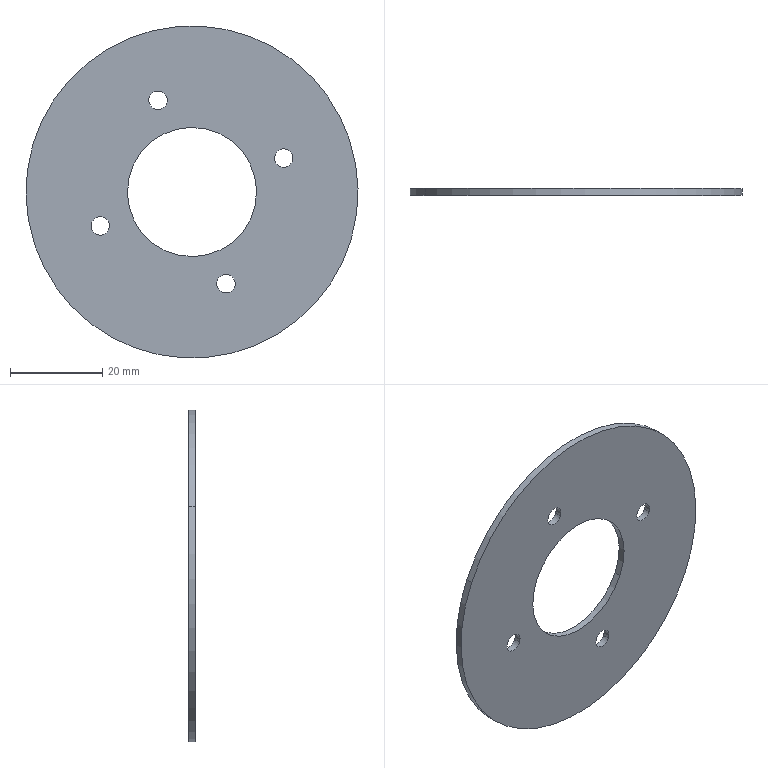Component | SolidWorks | Gear cover-1 | 1 solid | 14 faces | box 72 x 1.5 x 72 mm | volume 5108 mm3 | cylinder 12 | plane 2 | commonest cylinder face diameters 4 x8 28 x2 72 x2
STEP:
#1=COLOUR_RGB('',0.7922,0.8196,0.9333);
#2=FILL_AREA_STYLE_COLOUR('',#1);
#3=FILL_AREA_STYLE('',(#2));
#4=SURFACE_STYLE_FILL_AREA(#3);
#5=SURFACE_SIDE_STYLE('',(#4));
#6=SURFACE_STYLE_USAGE(.BOTH.,#5);
#7=PRESENTATION_STYLE_ASSIGNMENT((#6));
#8=CARTESIAN_POINT('',(-1.289,-1.213,-2.141));
#9=VERTEX_POINT('',#8);
#10=CARTESIAN_POINT('',(-1.146,-1.213,-2.207));
#11=VERTEX_POINT('',#10);
#12=CARTESIAN_POINT('',(-1.218,-1.213,-2.174));
#13=DIRECTION('',(-0.,-1.,0.));
#14=DIRECTION('',(0.9087,0.,-0.4174));
#15=AXIS2_PLACEMENT_3D('',#12,#13,#14);
#16=CIRCLE('',#15,0.07874);
#17=EDGE_CURVE('',#9,#11,#16,.T.);
#18=ORIENTED_EDGE('',*,*,#17,.T.);
#19=CARTESIAN_POINT('',(-1.146,-1.154,-2.207));
#20=VERTEX_POINT('',#19);
#21=CARTESIAN_POINT('',(-1.146,-1.213,-2.207));
#22=DIRECTION('',(0.,1.,-0.));
#23=VECTOR('',#22,39.37);
#24=LINE('',#21,#23);
#25=EDGE_CURVE('',#11,#20,#24,.T.);
#26=ORIENTED_EDGE('',*,*,#25,.T.);
#27=CARTESIAN_POINT('',(-1.289,-1.154,-2.141));
#28=VERTEX_POINT('',#27);
#29=CARTESIAN_POINT('',(-1.218,-1.154,-2.174));
#30=DIRECTION('',(-0.,-1.,0.));
#31=DIRECTION('',(0.9087,0.,-0.4174));
#32=AXIS2_PLACEMENT_3D('',#29,#30,#31);
#33=CIRCLE('',#32,0.07874);
#34=EDGE_CURVE('',#28,#20,#33,.T.);
#35=ORIENTED_EDGE('',*,*,#34,.F.);
#36=CARTESIAN_POINT('',(-1.289,-1.213,-2.141));
#37=DIRECTION('',(0.,1.,-0.));
#38=VECTOR('',#37,39.37);
#39=LINE('',#36,#38);
#40=EDGE_CURVE('',#9,#28,#39,.T.);
#41=ORIENTED_EDGE('',*,*,#40,.F.);
#42=EDGE_LOOP('',(#18,#26,#35,#41));
#43=FACE_OUTER_BOUND('',#42,.T.);
#44=CARTESIAN_POINT('',(-1.218,-1.213,-2.174));
#45=DIRECTION('',(0.,1.,-0.));
#46=DIRECTION('',(-0.9087,0.,0.4174));
#47=AXIS2_PLACEMENT_3D('',#44,#45,#46);
#48=CYLINDRICAL_SURFACE('',#47,0.07874);
#49=ADVANCED_FACE('',(#43),#48,.F.);
#50=CARTESIAN_POINT('',(-0.216,-1.213,-2.634));
#51=VERTEX_POINT('',#50);
#52=CARTESIAN_POINT('',(-0.0729,-1.213,-2.7));
#53=VERTEX_POINT('',#52);
#54=CARTESIAN_POINT('',(-0.1445,-1.213,-2.667));
#55=DIRECTION('',(-0.,-1.,0.));
#56=DIRECTION('',(0.9087,0.,-0.4174));
#57=AXIS2_PLACEMENT_3D('',#54,#55,#56);
#58=CIRCLE('',#57,0.07874);
#59=EDGE_CURVE('',#51,#53,#58,.T.);
#60=ORIENTED_EDGE('',*,*,#59,.T.);
#61=CARTESIAN_POINT('',(-0.0729,-1.154,-2.7));
#62=VERTEX_POINT('',#61);
#63=CARTESIAN_POINT('',(-0.0729,-1.213,-2.7));
#64=DIRECTION('',(0.,1.,-0.));
#65=VECTOR('',#64,39.37);
#66=LINE('',#63,#65);
#67=EDGE_CURVE('',#53,#62,#66,.T.);
#68=ORIENTED_EDGE('',*,*,#67,.T.);
#69=CARTESIAN_POINT('',(-0.216,-1.154,-2.634));
#70=VERTEX_POINT('',#69);
#71=CARTESIAN_POINT('',(-0.1445,-1.154,-2.667));
#72=DIRECTION('',(-0.,-1.,0.));
#73=DIRECTION('',(0.9087,0.,-0.4174));
#74=AXIS2_PLACEMENT_3D('',#71,#72,#73);
#75=CIRCLE('',#74,0.07874);
#76=EDGE_CURVE('',#70,#62,#75,.T.);
#77=ORIENTED_EDGE('',*,*,#76,.F.);
#78=CARTESIAN_POINT('',(-0.216,-1.213,-2.634));
#79=DIRECTION('',(0.,1.,-0.));
#80=VECTOR('',#79,39.37);
#81=LINE('',#78,#80);
#82=EDGE_CURVE('',#51,#70,#81,.T.);
#83=ORIENTED_EDGE('',*,*,#82,.F.);
#84=EDGE_LOOP('',(#60,#68,#77,#83));
#85=FACE_OUTER_BOUND('',#84,.T.);
#86=CARTESIAN_POINT('',(-0.1445,-1.213,-2.667));
#87=DIRECTION('',(0.,1.,-0.));
#88=DIRECTION('',(-0.9087,0.,0.4174));
#89=AXIS2_PLACEMENT_3D('',#86,#87,#88);
#90=CYLINDRICAL_SURFACE('',#89,0.07874);
#91=ADVANCED_FACE('',(#85),#90,.F.);
#92=CARTESIAN_POINT('',(0.277,-1.213,-1.561));
#93=VERTEX_POINT('',#92);
#94=CARTESIAN_POINT('',(0.4201,-1.213,-1.627));
#95=VERTEX_POINT('',#94);
#96=CARTESIAN_POINT('',(0.3486,-1.213,-1.594));
#97=DIRECTION('',(-0.,-1.,0.));
#98=DIRECTION('',(0.9087,0.,-0.4174));
#99=AXIS2_PLACEMENT_3D('',#96,#97,#98);
#100=CIRCLE('',#99,0.07874);
#101=EDGE_CURVE('',#93,#95,#100,.T.);
#102=ORIENTED_EDGE('',*,*,#101,.T.);
#103=CARTESIAN_POINT('',(0.4201,-1.154,-1.627));
#104=VERTEX_POINT('',#103);
#105=CARTESIAN_POINT('',(0.4201,-1.213,-1.627));
#106=DIRECTION('',(0.,1.,-0.));
#107=VECTOR('',#106,39.37);
#108=LINE('',#105,#107);
#109=EDGE_CURVE('',#95,#104,#108,.T.);
#110=ORIENTED_EDGE('',*,*,#109,.T.);
#111=CARTESIAN_POINT('',(0.277,-1.154,-1.561));
#112=VERTEX_POINT('',#111);
#113=CARTESIAN_POINT('',(0.3486,-1.154,-1.594));
#114=DIRECTION('',(-0.,-1.,0.));
#115=DIRECTION('',(0.9087,0.,-0.4174));
#116=AXIS2_PLACEMENT_3D('',#113,#114,#115);
#117=CIRCLE('',#116,0.07874);
#118=EDGE_CURVE('',#112,#104,#117,.T.);
#119=ORIENTED_EDGE('',*,*,#118,.F.);
#120=CARTESIAN_POINT('',(0.277,-1.213,-1.561));
#121=DIRECTION('',(0.,1.,-0.));
#122=VECTOR('',#121,39.37);
#123=LINE('',#120,#122);
#124=EDGE_CURVE('',#93,#112,#123,.T.);
#125=ORIENTED_EDGE('',*,*,#124,.F.);
#126=EDGE_LOOP('',(#102,#110,#119,#125));
#127=FACE_OUTER_BOUND('',#126,.T.);
#128=CARTESIAN_POINT('',(0.3486,-1.213,-1.594));
#129=DIRECTION('',(0.,1.,-0.));
#130=DIRECTION('',(-0.9087,0.,0.4174));
#131=AXIS2_PLACEMENT_3D('',#128,#129,#130);
#132=CYLINDRICAL_SURFACE('',#131,0.07874);
#133=ADVANCED_FACE('',(#127),#132,.F.);
#134=CARTESIAN_POINT('',(-0.7963,-1.213,-1.068));
#135=VERTEX_POINT('',#134);
#136=CARTESIAN_POINT('',(-0.6532,-1.213,-1.134));
#137=VERTEX_POINT('',#136);
#138=CARTESIAN_POINT('',(-0.7247,-1.213,-1.101));
#139=DIRECTION('',(-0.,-1.,0.));
#140=DIRECTION('',(0.9087,0.,-0.4174));
#141=AXIS2_PLACEMENT_3D('',#138,#139,#140);
#142=CIRCLE('',#141,0.07874);
#143=EDGE_CURVE('',#135,#137,#142,.T.);
#144=ORIENTED_EDGE('',*,*,#143,.T.);
#145=CARTESIAN_POINT('',(-0.6532,-1.154,-1.134));
#146=VERTEX_POINT('',#145);
#147=CARTESIAN_POINT('',(-0.6532,-1.213,-1.134));
#148=DIRECTION('',(0.,1.,-0.));
#149=VECTOR('',#148,39.37);
#150=LINE('',#147,#149);
#151=EDGE_CURVE('',#137,#146,#150,.T.);
#152=ORIENTED_EDGE('',*,*,#151,.T.);
#153=CARTESIAN_POINT('',(-0.7963,-1.154,-1.068));
#154=VERTEX_POINT('',#153);
#155=CARTESIAN_POINT('',(-0.7247,-1.154,-1.101));
#156=DIRECTION('',(-0.,-1.,0.));
#157=DIRECTION('',(0.9087,0.,-0.4174));
#158=AXIS2_PLACEMENT_3D('',#155,#156,#157);
#159=CIRCLE('',#158,0.07874);
#160=EDGE_CURVE('',#154,#146,#159,.T.);
#161=ORIENTED_EDGE('',*,*,#160,.F.);
#162=CARTESIAN_POINT('',(-0.7963,-1.213,-1.068));
#163=DIRECTION('',(0.,1.,-0.));
#164=VECTOR('',#163,39.37);
#165=LINE('',#162,#164);
#166=EDGE_CURVE('',#135,#154,#165,.T.);
#167=ORIENTED_EDGE('',*,*,#166,.F.);
#168=EDGE_LOOP('',(#144,#152,#161,#167));
#169=FACE_OUTER_BOUND('',#168,.T.);
#170=CARTESIAN_POINT('',(-0.7247,-1.213,-1.101));
#171=DIRECTION('',(0.,1.,-0.));
#172=DIRECTION('',(-0.9087,0.,0.4174));
#173=AXIS2_PLACEMENT_3D('',#170,#171,#172);
#174=CYLINDRICAL_SURFACE('',#173,0.07874);
#175=ADVANCED_FACE('',(#169),#174,.F.);
#176=CARTESIAN_POINT('',(-0.9354,-1.213,-1.654));
#177=VERTEX_POINT('',#176);
#178=CARTESIAN_POINT('',(0.06628,-1.213,-2.114));
#179=VERTEX_POINT('',#178);
#180=CARTESIAN_POINT('',(-0.4346,-1.213,-1.884));
#181=DIRECTION('',(-0.,-1.,0.));
#182=DIRECTION('',(0.9087,-0.,-0.4174));
#183=AXIS2_PLACEMENT_3D('',#180,#181,#182);
#184=CIRCLE('',#183,0.5512);
#185=EDGE_CURVE('',#177,#179,#184,.T.);
#186=ORIENTED_EDGE('',*,*,#185,.T.);
#187=CARTESIAN_POINT('',(0.06628,-1.154,-2.114));
#188=VERTEX_POINT('',#187);
#189=CARTESIAN_POINT('',(0.06628,-1.213,-2.114));
#190=DIRECTION('',(0.,1.,-0.));
#191=VECTOR('',#190,39.37);
#192=LINE('',#189,#191);
#193=EDGE_CURVE('',#179,#188,#192,.T.);
#194=ORIENTED_EDGE('',*,*,#193,.T.);
#195=CARTESIAN_POINT('',(-0.9354,-1.154,-1.654));
#196=VERTEX_POINT('',#195);
#197=CARTESIAN_POINT('',(-0.4346,-1.154,-1.884));
#198=DIRECTION('',(-0.,-1.,0.));
#199=DIRECTION('',(0.9087,-0.,-0.4174));
#200=AXIS2_PLACEMENT_3D('',#197,#198,#199);
#201=CIRCLE('',#200,0.5512);
#202=EDGE_CURVE('',#196,#188,#201,.T.);
#203=ORIENTED_EDGE('',*,*,#202,.F.);
#204=CARTESIAN_POINT('',(-0.9354,-1.213,-1.654));
#205=DIRECTION('',(0.,1.,-0.));
#206=VECTOR('',#205,39.37);
#207=LINE('',#204,#206);
#208=EDGE_CURVE('',#177,#196,#207,.T.);
#209=ORIENTED_EDGE('',*,*,#208,.F.);
#210=EDGE_LOOP('',(#186,#194,#203,#209));
#211=FACE_OUTER_BOUND('',#210,.T.);
#212=CARTESIAN_POINT('',(-0.4346,-1.213,-1.884));
#213=DIRECTION('',(0.,1.,-0.));
#214=DIRECTION('',(-0.9087,0.,0.4174));
#215=AXIS2_PLACEMENT_3D('',#212,#213,#214);
#216=CYLINDRICAL_SURFACE('',#215,0.5512);
#217=ADVANCED_FACE('',(#211),#216,.F.);
#218=CARTESIAN_POINT('',(0.8534,-1.213,-2.476));
#219=VERTEX_POINT('',#218);
#220=CARTESIAN_POINT('',(-1.723,-1.213,-1.292));
#221=VERTEX_POINT('',#220);
#222=CARTESIAN_POINT('',(-0.4346,-1.213,-1.884));
#223=DIRECTION('',(-0.,-1.,0.));
#224=DIRECTION('',(0.9087,-0.,-0.4174));
#225=AXIS2_PLACEMENT_3D('',#222,#223,#224);
#226=CIRCLE('',#225,1.417);
#227=EDGE_CURVE('',#219,#221,#226,.T.);
#228=ORIENTED_EDGE('',*,*,#227,.F.);
#229=CARTESIAN_POINT('',(0.8534,-1.154,-2.476));
#230=VERTEX_POINT('',#229);
#231=CARTESIAN_POINT('',(0.8534,-1.213,-2.476));
#232=DIRECTION('',(0.,1.,-0.));
#233=VECTOR('',#232,39.37);
#234=LINE('',#231,#233);
#235=EDGE_CURVE('',#219,#230,#234,.T.);
#236=ORIENTED_EDGE('',*,*,#235,.T.);
#237=CARTESIAN_POINT('',(-1.723,-1.154,-1.292));
#238=VERTEX_POINT('',#237);
#239=CARTESIAN_POINT('',(-0.4346,-1.154,-1.884));
#240=DIRECTION('',(-0.,-1.,0.));
#241=DIRECTION('',(0.9087,-0.,-0.4174));
#242=AXIS2_PLACEMENT_3D('',#239,#240,#241);
#243=CIRCLE('',#242,1.417);
#244=EDGE_CURVE('',#230,#238,#243,.T.);
#245=ORIENTED_EDGE('',*,*,#244,.T.);
#246=CARTESIAN_POINT('',(-1.723,-1.213,-1.292));
#247=DIRECTION('',(0.,1.,-0.));
#248=VECTOR('',#247,39.37);
#249=LINE('',#246,#248);
#250=EDGE_CURVE('',#221,#238,#249,.T.);
#251=ORIENTED_EDGE('',*,*,#250,.F.);
#252=EDGE_LOOP('',(#228,#236,#245,#251));
#253=FACE_OUTER_BOUND('',#252,.T.);
#254=CARTESIAN_POINT('',(-0.4346,-1.213,-1.884));
#255=DIRECTION('',(0.,1.,-0.));
#256=DIRECTION('',(-0.9087,0.,0.4174));
#257=AXIS2_PLACEMENT_3D('',#254,#255,#256);
#258=CYLINDRICAL_SURFACE('',#257,1.417);
#259=ADVANCED_FACE('',(#253),#258,.T.);
#260=ORIENTED_EDGE('',*,*,#59,.F.);
#261=CARTESIAN_POINT('',(-0.1445,-1.213,-2.667));
#262=DIRECTION('',(-0.,-1.,0.));
#263=DIRECTION('',(0.9087,0.,-0.4174));
#264=AXIS2_PLACEMENT_3D('',#261,#262,#263);
#265=CIRCLE('',#264,0.07874);
#266=EDGE_CURVE('',#53,#51,#265,.T.);
#267=ORIENTED_EDGE('',*,*,#266,.F.);
#268=EDGE_LOOP('',(#260,#267));
#269=FACE_BOUND('',#268,.T.);
#270=ORIENTED_EDGE('',*,*,#143,.F.);
#271=CARTESIAN_POINT('',(-0.7247,-1.213,-1.101));
#272=DIRECTION('',(-0.,-1.,0.));
#273=DIRECTION('',(0.9087,0.,-0.4174));
#274=AXIS2_PLACEMENT_3D('',#271,#272,#273);
#275=CIRCLE('',#274,0.07874);
#276=EDGE_CURVE('',#137,#135,#275,.T.);
#277=ORIENTED_EDGE('',*,*,#276,.F.);
#278=EDGE_LOOP('',(#270,#277));
#279=FACE_BOUND('',#278,.T.);
#280=CARTESIAN_POINT('',(-0.4346,-1.213,-1.884));
#281=DIRECTION('',(-0.,-1.,0.));
#282=DIRECTION('',(0.9087,-0.,-0.4174));
#283=AXIS2_PLACEMENT_3D('',#280,#281,#282);
#284=CIRCLE('',#283,1.417);
#285=EDGE_CURVE('',#221,#219,#284,.T.);
#286=ORIENTED_EDGE('',*,*,#285,.T.);
#287=ORIENTED_EDGE('',*,*,#227,.T.);
#288=EDGE_LOOP('',(#286,#287));
#289=FACE_OUTER_BOUND('',#288,.T.);
#290=ORIENTED_EDGE('',*,*,#185,.F.);
#291=CARTESIAN_POINT('',(-0.4346,-1.213,-1.884));
#292=DIRECTION('',(-0.,-1.,0.));
#293=DIRECTION('',(0.9087,-0.,-0.4174));
#294=AXIS2_PLACEMENT_3D('',#291,#292,#293);
#295=CIRCLE('',#294,0.5512);
#296=EDGE_CURVE('',#179,#177,#295,.T.);
#297=ORIENTED_EDGE('',*,*,#296,.F.);
#298=EDGE_LOOP('',(#290,#297));
#299=FACE_BOUND('',#298,.T.);
#300=ORIENTED_EDGE('',*,*,#101,.F.);
#301=CARTESIAN_POINT('',(0.3486,-1.213,-1.594));
#302=DIRECTION('',(-0.,-1.,0.));
#303=DIRECTION('',(0.9087,0.,-0.4174));
#304=AXIS2_PLACEMENT_3D('',#301,#302,#303);
#305=CIRCLE('',#304,0.07874);
#306=EDGE_CURVE('',#95,#93,#305,.T.);
#307=ORIENTED_EDGE('',*,*,#306,.F.);
#308=EDGE_LOOP('',(#300,#307));
#309=FACE_BOUND('',#308,.T.);
#310=ORIENTED_EDGE('',*,*,#17,.F.);
#311=CARTESIAN_POINT('',(-1.218,-1.213,-2.174));
#312=DIRECTION('',(-0.,-1.,0.));
#313=DIRECTION('',(0.9087,0.,-0.4174));
#314=AXIS2_PLACEMENT_3D('',#311,#312,#313);
#315=CIRCLE('',#314,0.07874);
#316=EDGE_CURVE('',#11,#9,#315,.T.);
#317=ORIENTED_EDGE('',*,*,#316,.F.);
#318=EDGE_LOOP('',(#310,#317));
#319=FACE_BOUND('',#318,.T.);
#320=CARTESIAN_POINT('',(-0.4346,-1.213,-1.884));
#321=DIRECTION('',(-0.,-1.,0.));
#322=DIRECTION('',(0.9087,-0.,-0.4174));
#323=AXIS2_PLACEMENT_3D('',#320,#321,#322);
#324=PLANE('',#323);
#325=ADVANCED_FACE('',(#269,#279,#289,#299,#309,#319),#324,.T.);
#326=ORIENTED_EDGE('',*,*,#76,.T.);
#327=CARTESIAN_POINT('',(-0.1445,-1.154,-2.667));
#328=DIRECTION('',(-0.,-1.,0.));
#329=DIRECTION('',(0.9087,0.,-0.4174));
#330=AXIS2_PLACEMENT_3D('',#327,#328,#329);
#331=CIRCLE('',#330,0.07874);
#332=EDGE_CURVE('',#62,#70,#331,.T.);
#333=ORIENTED_EDGE('',*,*,#332,.T.);
#334=EDGE_LOOP('',(#326,#333));
#335=FACE_BOUND('',#334,.T.);
#336=ORIENTED_EDGE('',*,*,#160,.T.);
#337=CARTESIAN_POINT('',(-0.7247,-1.154,-1.101));
#338=DIRECTION('',(-0.,-1.,0.));
#339=DIRECTION('',(0.9087,0.,-0.4174));
#340=AXIS2_PLACEMENT_3D('',#337,#338,#339);
#341=CIRCLE('',#340,0.07874);
#342=EDGE_CURVE('',#146,#154,#341,.T.);
#343=ORIENTED_EDGE('',*,*,#342,.T.);
#344=EDGE_LOOP('',(#336,#343));
#345=FACE_BOUND('',#344,.T.);
#346=CARTESIAN_POINT('',(-0.4346,-1.154,-1.884));
#347=DIRECTION('',(-0.,-1.,0.));
#348=DIRECTION('',(0.9087,-0.,-0.4174));
#349=AXIS2_PLACEMENT_3D('',#346,#347,#348);
#350=CIRCLE('',#349,1.417);
#351=EDGE_CURVE('',#238,#230,#350,.T.);
#352=ORIENTED_EDGE('',*,*,#351,.F.);
#353=ORIENTED_EDGE('',*,*,#244,.F.);
#354=EDGE_LOOP('',(#352,#353));
#355=FACE_OUTER_BOUND('',#354,.T.);
#356=ORIENTED_EDGE('',*,*,#202,.T.);
#357=CARTESIAN_POINT('',(-0.4346,-1.154,-1.884));
#358=DIRECTION('',(-0.,-1.,0.));
#359=DIRECTION('',(0.9087,-0.,-0.4174));
#360=AXIS2_PLACEMENT_3D('',#357,#358,#359);
#361=CIRCLE('',#360,0.5512);
#362=EDGE_CURVE('',#188,#196,#361,.T.);
#363=ORIENTED_EDGE('',*,*,#362,.T.);
#364=EDGE_LOOP('',(#356,#363));
#365=FACE_BOUND('',#364,.T.);
#366=ORIENTED_EDGE('',*,*,#118,.T.);
#367=CARTESIAN_POINT('',(0.3486,-1.154,-1.594));
#368=DIRECTION('',(-0.,-1.,0.));
#369=DIRECTION('',(0.9087,0.,-0.4174));
#370=AXIS2_PLACEMENT_3D('',#367,#368,#369);
#371=CIRCLE('',#370,0.07874);
#372=EDGE_CURVE('',#104,#112,#371,.T.);
#373=ORIENTED_EDGE('',*,*,#372,.T.);
#374=EDGE_LOOP('',(#366,#373));
#375=FACE_BOUND('',#374,.T.);
#376=ORIENTED_EDGE('',*,*,#34,.T.);
#377=CARTESIAN_POINT('',(-1.218,-1.154,-2.174));
#378=DIRECTION('',(-0.,-1.,0.));
#379=DIRECTION('',(0.9087,0.,-0.4174));
#380=AXIS2_PLACEMENT_3D('',#377,#378,#379);
#381=CIRCLE('',#380,0.07874);
#382=EDGE_CURVE('',#20,#28,#381,.T.);
#383=ORIENTED_EDGE('',*,*,#382,.T.);
#384=EDGE_LOOP('',(#376,#383));
#385=FACE_BOUND('',#384,.T.);
#386=CARTESIAN_POINT('',(-0.4346,-1.154,-1.884));
#387=DIRECTION('',(-0.,-1.,0.));
#388=DIRECTION('',(0.9087,-0.,-0.4174));
#389=AXIS2_PLACEMENT_3D('',#386,#387,#388);
#390=PLANE('',#389);
#391=ADVANCED_FACE('',(#335,#345,#355,#365,#375,#385),#390,.F.);
#392=ORIENTED_EDGE('',*,*,#235,.F.);
#393=ORIENTED_EDGE('',*,*,#285,.F.);
#394=ORIENTED_EDGE('',*,*,#250,.T.);
#395=ORIENTED_EDGE('',*,*,#351,.T.);
#396=EDGE_LOOP('',(#392,#393,#394,#395));
#397=FACE_OUTER_BOUND('',#396,.T.);
#398=CARTESIAN_POINT('',(-0.4346,-1.213,-1.884));
#399=DIRECTION('',(0.,1.,-0.));
#400=DIRECTION('',(-0.9087,0.,0.4174));
#401=AXIS2_PLACEMENT_3D('',#398,#399,#400);
#402=CYLINDRICAL_SURFACE('',#401,1.417);
#403=ADVANCED_FACE('',(#397),#402,.T.);
#404=ORIENTED_EDGE('',*,*,#193,.F.);
#405=ORIENTED_EDGE('',*,*,#296,.T.);
#406=ORIENTED_EDGE('',*,*,#208,.T.);
#407=ORIENTED_EDGE('',*,*,#362,.F.);
#408=EDGE_LOOP('',(#404,#405,#406,#407));
#409=FACE_OUTER_BOUND('',#408,.T.);
#410=CARTESIAN_POINT('',(-0.4346,-1.213,-1.884));
#411=DIRECTION('',(0.,1.,-0.));
#412=DIRECTION('',(-0.9087,0.,0.4174));
#413=AXIS2_PLACEMENT_3D('',#410,#411,#412);
#414=CYLINDRICAL_SURFACE('',#413,0.5512);
#415=ADVANCED_FACE('',(#409),#414,.F.);
#416=ORIENTED_EDGE('',*,*,#151,.F.);
#417=ORIENTED_EDGE('',*,*,#276,.T.);
#418=ORIENTED_EDGE('',*,*,#166,.T.);
#419=ORIENTED_EDGE('',*,*,#342,.F.);
#420=EDGE_LOOP('',(#416,#417,#418,#419));
#421=FACE_OUTER_BOUND('',#420,.T.);
#422=CARTESIAN_POINT('',(-0.7247,-1.213,-1.101));
#423=DIRECTION('',(0.,1.,-0.));
#424=DIRECTION('',(-0.9087,0.,0.4174));
#425=AXIS2_PLACEMENT_3D('',#422,#423,#424);
#426=CYLINDRICAL_SURFACE('',#425,0.07874);
#427=ADVANCED_FACE('',(#421),#426,.F.);
#428=ORIENTED_EDGE('',*,*,#109,.F.);
#429=ORIENTED_EDGE('',*,*,#306,.T.);
#430=ORIENTED_EDGE('',*,*,#124,.T.);
#431=ORIENTED_EDGE('',*,*,#372,.F.);
#432=EDGE_LOOP('',(#428,#429,#430,#431));
#433=FACE_OUTER_BOUND('',#432,.T.);
#434=CARTESIAN_POINT('',(0.3486,-1.213,-1.594));
#435=DIRECTION('',(0.,1.,-0.));
#436=DIRECTION('',(-0.9087,0.,0.4174));
#437=AXIS2_PLACEMENT_3D('',#434,#435,#436);
#438=CYLINDRICAL_SURFACE('',#437,0.07874);
#439=ADVANCED_FACE('',(#433),#438,.F.);
#440=ORIENTED_EDGE('',*,*,#67,.F.);
#441=ORIENTED_EDGE('',*,*,#266,.T.);
#442=ORIENTED_EDGE('',*,*,#82,.T.);
#443=ORIENTED_EDGE('',*,*,#332,.F.);
#444=EDGE_LOOP('',(#440,#441,#442,#443));
#445=FACE_OUTER_BOUND('',#444,.T.);
#446=CARTESIAN_POINT('',(-0.1445,-1.213,-2.667));
#447=DIRECTION('',(0.,1.,-0.));
#448=DIRECTION('',(-0.9087,0.,0.4174));
#449=AXIS2_PLACEMENT_3D('',#446,#447,#448);
#450=CYLINDRICAL_SURFACE('',#449,0.07874);
#451=ADVANCED_FACE('',(#445),#450,.F.);
#452=ORIENTED_EDGE('',*,*,#25,.F.);
#453=ORIENTED_EDGE('',*,*,#316,.T.);
#454=ORIENTED_EDGE('',*,*,#40,.T.);
#455=ORIENTED_EDGE('',*,*,#382,.F.);
#456=EDGE_LOOP('',(#452,#453,#454,#455));
#457=FACE_OUTER_BOUND('',#456,.T.);
#458=CARTESIAN_POINT('',(-1.218,-1.213,-2.174));
#459=DIRECTION('',(0.,1.,-0.));
#460=DIRECTION('',(-0.9087,0.,0.4174));
#461=AXIS2_PLACEMENT_3D('',#458,#459,#460);
#462=CYLINDRICAL_SURFACE('',#461,0.07874);
#463=ADVANCED_FACE('',(#457),#462,.F.);
#464=CLOSED_SHELL('',(#49,#91,#133,#175,#217,#259,#325,#391,#403,#415,#427,#439,#451,#463));
#465=MANIFOLD_SOLID_BREP('',#464);
#466=STYLED_ITEM('',(#7),#465);
#467=PRESENTATION_LAYER_ASSIGNMENT('','',(#466));
#468=(LENGTH_UNIT()NAMED_UNIT(*)SI_UNIT($,.METRE.));
#469=LENGTH_MEASURE_WITH_UNIT(LENGTH_MEASURE(0.0254),#468);
#470=DIMENSIONAL_EXPONENTS(1.,0.,0.,0.,0.,0.,0.);
#471=(CONVERSION_BASED_UNIT('',#469)LENGTH_UNIT()NAMED_UNIT(#470));
#472=UNCERTAINTY_MEASURE_WITH_UNIT(LENGTH_MEASURE(0.00001),#471,'','');
#473=(NAMED_UNIT(*)PLANE_ANGLE_UNIT()SI_UNIT($,.RADIAN.));
#474=(NAMED_UNIT(*)SI_UNIT($,.STERADIAN.)SOLID_ANGLE_UNIT());
#475=(GEOMETRIC_REPRESENTATION_CONTEXT(3)GLOBAL_UNCERTAINTY_ASSIGNED_CONTEXT((#472))GLOBAL_UNIT_ASSIGNED_CONTEXT((#471,#473,#474))REPRESENTATION_CONTEXT('',''));
#476=MECHANICAL_DESIGN_GEOMETRIC_PRESENTATION_REPRESENTATION('',(#466),#475);
#477=CARTESIAN_POINT('',(0.,0.,0.));
#478=DIRECTION('',(0.,0.,1.));
#479=DIRECTION('',(1.,0.,0.));
#480=AXIS2_PLACEMENT_3D('',#477,#478,#479);
#481=(LENGTH_UNIT()NAMED_UNIT(*)SI_UNIT($,.METRE.));
#482=LENGTH_MEASURE_WITH_UNIT(LENGTH_MEASURE(0.0254),#481);
#483=DIMENSIONAL_EXPONENTS(1.,0.,0.,0.,0.,0.,0.);
#484=(CONVERSION_BASED_UNIT('',#482)LENGTH_UNIT()NAMED_UNIT(#483));
#485=UNCERTAINTY_MEASURE_WITH_UNIT(LENGTH_MEASURE(0.00001),#484,'','');
#486=(NAMED_UNIT(*)PLANE_ANGLE_UNIT()SI_UNIT($,.RADIAN.));
#487=(NAMED_UNIT(*)SI_UNIT($,.STERADIAN.)SOLID_ANGLE_UNIT());
#488=(GEOMETRIC_REPRESENTATION_CONTEXT(3)GLOBAL_UNCERTAINTY_ASSIGNED_CONTEXT((#485))GLOBAL_UNIT_ASSIGNED_CONTEXT((#484,#486,#487))REPRESENTATION_CONTEXT('',''));
#489=ADVANCED_BREP_SHAPE_REPRESENTATION('',(#465,#480),#488);